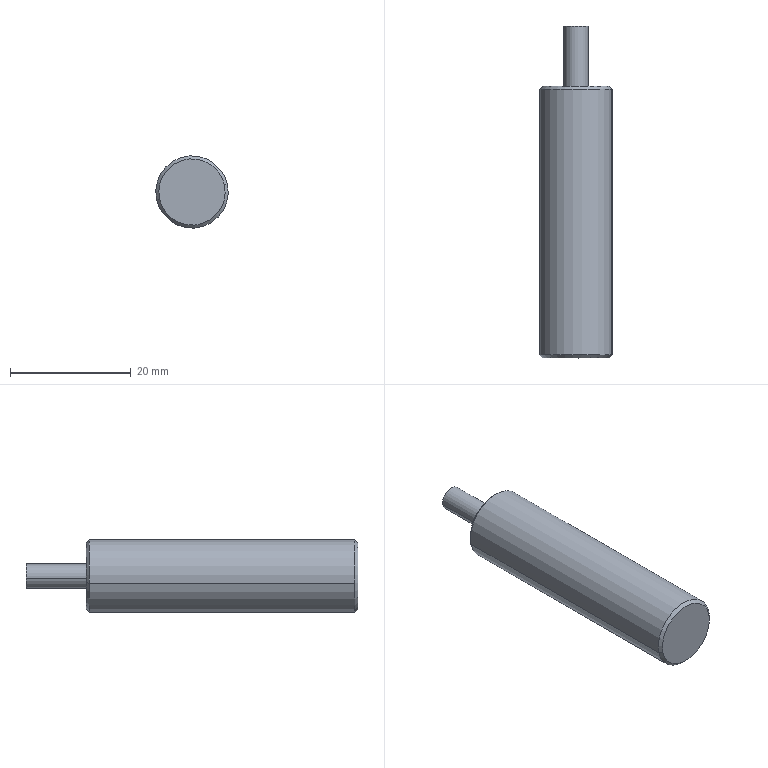Component | SolidWorks | ZJG28-1 | 1 solid | 11 faces | box 12 x 55 x 12 mm | volume 5206 mm3 | cone 4 | cylinder 4 | plane 3 | commonest cylinder face diameters 4 x2 12 x2
build123d program:
from build123d import *

# Parameters (mm, degrees)
SKETCH1_R           = 6
BOSS_EXTRUDE1_DEPTH = 45
SKETCH2_R           = 2
BOSS_EXTRUDE2_DEPTH = 10
CHAMFER1_SIZE       = 0.5


with BuildPart() as part:
    # Sketch1 → Boss-Extrude1 (new body)
    with BuildSketch(Plane.XY):
        with Locations(Location((0, 0, 0), (0, 0, 180))):
            Circle(SKETCH1_R)
    extrude(amount=BOSS_EXTRUDE1_DEPTH)

    # Sketch2 → Boss-Extrude2 (add)
    with BuildSketch(Plane.XY.offset(45)):
        Circle(SKETCH2_R)
    extrude(amount=BOSS_EXTRUDE2_DEPTH)

    # Chamfer1
    chamfer1_edges = [part.edges().sort_by_distance(p)[0] for p in [
        (6, 0, 0),
        (6, 0, 45),
    ]]
    chamfer(chamfer1_edges, length=CHAMFER1_SIZE)


solid = part.part

# Placed as in the assembly
solid = solid.moved(Location((-2.001, 46.001, -400), (-90, 0, 0)))
STEP:
#1=COLOUR_RGB('',0.7922,0.8196,0.9333);
#2=FILL_AREA_STYLE_COLOUR('',#1);
#3=FILL_AREA_STYLE('',(#2));
#4=SURFACE_STYLE_FILL_AREA(#3);
#5=SURFACE_SIDE_STYLE('',(#4));
#6=SURFACE_STYLE_USAGE(.BOTH.,#5);
#7=PRESENTATION_STYLE_ASSIGNMENT((#6));
#8=CARTESIAN_POINT('',(-0.2908,1.811,-15.792));
#9=VERTEX_POINT('',#8);
#10=CARTESIAN_POINT('',(0.1333,1.811,-15.704));
#11=VERTEX_POINT('',#10);
#12=CARTESIAN_POINT('',(-0.07876,1.811,-15.748));
#13=DIRECTION('',(0.,-1.,0.));
#14=DIRECTION('',(0.9793,0.,0.2022));
#15=AXIS2_PLACEMENT_3D('',#12,#13,#14);
#16=CIRCLE('',#15,0.2165);
#17=EDGE_CURVE('',#9,#11,#16,.T.);
#18=ORIENTED_EDGE('',*,*,#17,.F.);
#19=CARTESIAN_POINT('',(-0.3101,1.831,-15.796));
#20=VERTEX_POINT('',#19);
#21=CARTESIAN_POINT('',(-0.3101,1.831,-15.796));
#22=DIRECTION('',(-0.6925,0.7071,-0.143));
#23=VECTOR('',#22,39.37);
#24=LINE('',#21,#23);
#25=EDGE_CURVE('',#9,#20,#24,.T.);
#26=ORIENTED_EDGE('',*,*,#25,.T.);
#27=CARTESIAN_POINT('',(0.1526,1.831,-15.7));
#28=VERTEX_POINT('',#27);
#29=CARTESIAN_POINT('',(-0.07876,1.831,-15.748));
#30=DIRECTION('',(-0.,1.,-0.));
#31=DIRECTION('',(0.9793,0.,0.2022));
#32=AXIS2_PLACEMENT_3D('',#29,#30,#31);
#33=CIRCLE('',#32,0.2362);
#34=EDGE_CURVE('',#28,#20,#33,.T.);
#35=ORIENTED_EDGE('',*,*,#34,.F.);
#36=CARTESIAN_POINT('',(0.1526,1.831,-15.7));
#37=DIRECTION('',(0.6925,0.7071,0.143));
#38=VECTOR('',#37,39.37);
#39=LINE('',#36,#38);
#40=EDGE_CURVE('',#11,#28,#39,.T.);
#41=ORIENTED_EDGE('',*,*,#40,.F.);
#42=EDGE_LOOP('',(#18,#26,#35,#41));
#43=FACE_OUTER_BOUND('',#42,.T.);
#44=CARTESIAN_POINT('',(-0.07876,1.831,-15.748));
#45=DIRECTION('',(-0.,1.,-0.));
#46=DIRECTION('',(0.9793,0.,0.2022));
#47=AXIS2_PLACEMENT_3D('',#44,#45,#46);
#48=CONICAL_SURFACE('',#47,0.2362,0.7854);
#49=ADVANCED_FACE('',(#43),#48,.T.);
#50=CARTESIAN_POINT('',(0.1333,3.583,-15.704));
#51=VERTEX_POINT('',#50);
#52=CARTESIAN_POINT('',(-0.2908,3.583,-15.792));
#53=VERTEX_POINT('',#52);
#54=CARTESIAN_POINT('',(-0.07876,3.583,-15.748));
#55=DIRECTION('',(-0.,1.,-0.));
#56=DIRECTION('',(0.9793,0.,0.2022));
#57=AXIS2_PLACEMENT_3D('',#54,#55,#56);
#58=CIRCLE('',#57,0.2165);
#59=EDGE_CURVE('',#51,#53,#58,.T.);
#60=ORIENTED_EDGE('',*,*,#59,.F.);
#61=CARTESIAN_POINT('',(0.1526,3.563,-15.7));
#62=VERTEX_POINT('',#61);
#63=CARTESIAN_POINT('',(0.1333,3.583,-15.704));
#64=DIRECTION('',(0.6925,-0.7071,0.143));
#65=VECTOR('',#64,39.37);
#66=LINE('',#63,#65);
#67=EDGE_CURVE('',#51,#62,#66,.T.);
#68=ORIENTED_EDGE('',*,*,#67,.T.);
#69=CARTESIAN_POINT('',(-0.3101,3.563,-15.796));
#70=VERTEX_POINT('',#69);
#71=CARTESIAN_POINT('',(-0.07876,3.563,-15.748));
#72=DIRECTION('',(0.,-1.,0.));
#73=DIRECTION('',(0.9793,0.,0.2022));
#74=AXIS2_PLACEMENT_3D('',#71,#72,#73);
#75=CIRCLE('',#74,0.2362);
#76=EDGE_CURVE('',#70,#62,#75,.T.);
#77=ORIENTED_EDGE('',*,*,#76,.F.);
#78=CARTESIAN_POINT('',(-0.2908,3.583,-15.792));
#79=DIRECTION('',(-0.6925,-0.7071,-0.143));
#80=VECTOR('',#79,39.37);
#81=LINE('',#78,#80);
#82=EDGE_CURVE('',#53,#70,#81,.T.);
#83=ORIENTED_EDGE('',*,*,#82,.F.);
#84=EDGE_LOOP('',(#60,#68,#77,#83));
#85=FACE_OUTER_BOUND('',#84,.T.);
#86=CARTESIAN_POINT('',(-0.07876,3.583,-15.748));
#87=DIRECTION('',(0.,-1.,0.));
#88=DIRECTION('',(-0.9793,0.,-0.2022));
#89=AXIS2_PLACEMENT_3D('',#86,#87,#88);
#90=CONICAL_SURFACE('',#89,0.2165,0.7854);
#91=ADVANCED_FACE('',(#85),#90,.T.);
#92=CARTESIAN_POINT('',(-0.001647,3.976,-15.732));
#93=VERTEX_POINT('',#92);
#94=CARTESIAN_POINT('',(-0.1559,3.976,-15.764));
#95=VERTEX_POINT('',#94);
#96=CARTESIAN_POINT('',(-0.07876,3.976,-15.748));
#97=DIRECTION('',(-0.,1.,-0.));
#98=DIRECTION('',(0.9793,0.,0.2022));
#99=AXIS2_PLACEMENT_3D('',#96,#97,#98);
#100=CIRCLE('',#99,0.07874);
#101=EDGE_CURVE('',#93,#95,#100,.T.);
#102=ORIENTED_EDGE('',*,*,#101,.F.);
#103=CARTESIAN_POINT('',(-0.001647,3.583,-15.732));
#104=VERTEX_POINT('',#103);
#105=CARTESIAN_POINT('',(-0.001647,3.976,-15.732));
#106=DIRECTION('',(0.,-1.,0.));
#107=VECTOR('',#106,39.37);
#108=LINE('',#105,#107);
#109=EDGE_CURVE('',#93,#104,#108,.T.);
#110=ORIENTED_EDGE('',*,*,#109,.T.);
#111=CARTESIAN_POINT('',(-0.1559,3.583,-15.764));
#112=VERTEX_POINT('',#111);
#113=CARTESIAN_POINT('',(-0.07876,3.583,-15.748));
#114=DIRECTION('',(-0.,1.,-0.));
#115=DIRECTION('',(0.9793,0.,0.2022));
#116=AXIS2_PLACEMENT_3D('',#113,#114,#115);
#117=CIRCLE('',#116,0.07874);
#118=EDGE_CURVE('',#104,#112,#117,.T.);
#119=ORIENTED_EDGE('',*,*,#118,.T.);
#120=CARTESIAN_POINT('',(-0.1559,3.976,-15.764));
#121=DIRECTION('',(0.,-1.,0.));
#122=VECTOR('',#121,39.37);
#123=LINE('',#120,#122);
#124=EDGE_CURVE('',#95,#112,#123,.T.);
#125=ORIENTED_EDGE('',*,*,#124,.F.);
#126=EDGE_LOOP('',(#102,#110,#119,#125));
#127=FACE_OUTER_BOUND('',#126,.T.);
#128=CARTESIAN_POINT('',(-0.07876,3.976,-15.748));
#129=DIRECTION('',(0.,-1.,0.));
#130=DIRECTION('',(-0.9793,0.,-0.2022));
#131=AXIS2_PLACEMENT_3D('',#128,#129,#130);
#132=CYLINDRICAL_SURFACE('',#131,0.07874);
#133=ADVANCED_FACE('',(#127),#132,.T.);
#134=ORIENTED_EDGE('',*,*,#76,.T.);
#135=CARTESIAN_POINT('',(0.1526,3.583,-15.7));
#136=DIRECTION('',(0.,-1.,0.));
#137=VECTOR('',#136,39.37);
#138=LINE('',#135,#137);
#139=EDGE_CURVE('',#62,#28,#138,.T.);
#140=ORIENTED_EDGE('',*,*,#139,.T.);
#141=ORIENTED_EDGE('',*,*,#34,.T.);
#142=CARTESIAN_POINT('',(-0.3101,3.583,-15.796));
#143=DIRECTION('',(0.,-1.,0.));
#144=VECTOR('',#143,39.37);
#145=LINE('',#142,#144);
#146=EDGE_CURVE('',#70,#20,#145,.T.);
#147=ORIENTED_EDGE('',*,*,#146,.F.);
#148=EDGE_LOOP('',(#134,#140,#141,#147));
#149=FACE_OUTER_BOUND('',#148,.T.);
#150=CARTESIAN_POINT('',(-0.07876,3.583,-15.748));
#151=DIRECTION('',(0.,-1.,0.));
#152=DIRECTION('',(-0.9793,0.,-0.2022));
#153=AXIS2_PLACEMENT_3D('',#150,#151,#152);
#154=CYLINDRICAL_SURFACE('',#153,0.2362);
#155=ADVANCED_FACE('',(#149),#154,.T.);
#156=ORIENTED_EDGE('',*,*,#139,.F.);
#157=CARTESIAN_POINT('',(-0.07876,3.563,-15.748));
#158=DIRECTION('',(0.,-1.,0.));
#159=DIRECTION('',(0.9793,0.,0.2022));
#160=AXIS2_PLACEMENT_3D('',#157,#158,#159);
#161=CIRCLE('',#160,0.2362);
#162=EDGE_CURVE('',#62,#70,#161,.T.);
#163=ORIENTED_EDGE('',*,*,#162,.T.);
#164=ORIENTED_EDGE('',*,*,#146,.T.);
#165=CARTESIAN_POINT('',(-0.07876,1.831,-15.748));
#166=DIRECTION('',(-0.,1.,-0.));
#167=DIRECTION('',(0.9793,0.,0.2022));
#168=AXIS2_PLACEMENT_3D('',#165,#166,#167);
#169=CIRCLE('',#168,0.2362);
#170=EDGE_CURVE('',#20,#28,#169,.T.);
#171=ORIENTED_EDGE('',*,*,#170,.T.);
#172=EDGE_LOOP('',(#156,#163,#164,#171));
#173=FACE_OUTER_BOUND('',#172,.T.);
#174=CARTESIAN_POINT('',(-0.07876,3.583,-15.748));
#175=DIRECTION('',(0.,-1.,0.));
#176=DIRECTION('',(-0.9793,0.,-0.2022));
#177=AXIS2_PLACEMENT_3D('',#174,#175,#176);
#178=CYLINDRICAL_SURFACE('',#177,0.2362);
#179=ADVANCED_FACE('',(#173),#178,.T.);
#180=CARTESIAN_POINT('',(-0.07876,3.583,-15.748));
#181=DIRECTION('',(-0.,1.,-0.));
#182=DIRECTION('',(0.9793,0.,0.2022));
#183=AXIS2_PLACEMENT_3D('',#180,#181,#182);
#184=CIRCLE('',#183,0.2165);
#185=EDGE_CURVE('',#53,#51,#184,.T.);
#186=ORIENTED_EDGE('',*,*,#185,.T.);
#187=ORIENTED_EDGE('',*,*,#59,.T.);
#188=EDGE_LOOP('',(#186,#187));
#189=FACE_OUTER_BOUND('',#188,.T.);
#190=CARTESIAN_POINT('',(-0.07876,3.583,-15.748));
#191=DIRECTION('',(-0.,1.,-0.));
#192=DIRECTION('',(0.9793,0.,0.2022));
#193=AXIS2_PLACEMENT_3D('',#190,#191,#192);
#194=CIRCLE('',#193,0.07874);
#195=EDGE_CURVE('',#112,#104,#194,.T.);
#196=ORIENTED_EDGE('',*,*,#195,.F.);
#197=ORIENTED_EDGE('',*,*,#118,.F.);
#198=EDGE_LOOP('',(#196,#197));
#199=FACE_BOUND('',#198,.T.);
#200=CARTESIAN_POINT('',(-0.07876,3.583,-15.748));
#201=DIRECTION('',(-0.,1.,-0.));
#202=DIRECTION('',(0.9793,0.,0.2022));
#203=AXIS2_PLACEMENT_3D('',#200,#201,#202);
#204=PLANE('',#203);
#205=ADVANCED_FACE('',(#189,#199),#204,.T.);
#206=CARTESIAN_POINT('',(-0.07876,1.811,-15.748));
#207=DIRECTION('',(0.,-1.,0.));
#208=DIRECTION('',(0.9793,0.,0.2022));
#209=AXIS2_PLACEMENT_3D('',#206,#207,#208);
#210=CIRCLE('',#209,0.2165);
#211=EDGE_CURVE('',#11,#9,#210,.T.);
#212=ORIENTED_EDGE('',*,*,#211,.T.);
#213=ORIENTED_EDGE('',*,*,#17,.T.);
#214=EDGE_LOOP('',(#212,#213));
#215=FACE_OUTER_BOUND('',#214,.T.);
#216=CARTESIAN_POINT('',(-0.07876,1.811,-15.748));
#217=DIRECTION('',(-0.,1.,-0.));
#218=DIRECTION('',(0.9793,0.,0.2022));
#219=AXIS2_PLACEMENT_3D('',#216,#217,#218);
#220=PLANE('',#219);
#221=ADVANCED_FACE('',(#215),#220,.F.);
#222=ORIENTED_EDGE('',*,*,#109,.F.);
#223=CARTESIAN_POINT('',(-0.07876,3.976,-15.748));
#224=DIRECTION('',(-0.,1.,-0.));
#225=DIRECTION('',(0.9793,0.,0.2022));
#226=AXIS2_PLACEMENT_3D('',#223,#224,#225);
#227=CIRCLE('',#226,0.07874);
#228=EDGE_CURVE('',#95,#93,#227,.T.);
#229=ORIENTED_EDGE('',*,*,#228,.F.);
#230=ORIENTED_EDGE('',*,*,#124,.T.);
#231=ORIENTED_EDGE('',*,*,#195,.T.);
#232=EDGE_LOOP('',(#222,#229,#230,#231));
#233=FACE_OUTER_BOUND('',#232,.T.);
#234=CARTESIAN_POINT('',(-0.07876,3.976,-15.748));
#235=DIRECTION('',(0.,-1.,0.));
#236=DIRECTION('',(-0.9793,0.,-0.2022));
#237=AXIS2_PLACEMENT_3D('',#234,#235,#236);
#238=CYLINDRICAL_SURFACE('',#237,0.07874);
#239=ADVANCED_FACE('',(#233),#238,.T.);
#240=ORIENTED_EDGE('',*,*,#228,.T.);
#241=ORIENTED_EDGE('',*,*,#101,.T.);
#242=EDGE_LOOP('',(#240,#241));
#243=FACE_OUTER_BOUND('',#242,.T.);
#244=CARTESIAN_POINT('',(-0.07876,3.976,-15.748));
#245=DIRECTION('',(-0.,1.,-0.));
#246=DIRECTION('',(0.9793,0.,0.2022));
#247=AXIS2_PLACEMENT_3D('',#244,#245,#246);
#248=PLANE('',#247);
#249=ADVANCED_FACE('',(#243),#248,.T.);
#250=ORIENTED_EDGE('',*,*,#67,.F.);
#251=ORIENTED_EDGE('',*,*,#185,.F.);
#252=ORIENTED_EDGE('',*,*,#82,.T.);
#253=ORIENTED_EDGE('',*,*,#162,.F.);
#254=EDGE_LOOP('',(#250,#251,#252,#253));
#255=FACE_OUTER_BOUND('',#254,.T.);
#256=CARTESIAN_POINT('',(-0.07876,3.583,-15.748));
#257=DIRECTION('',(0.,-1.,0.));
#258=DIRECTION('',(-0.9793,0.,-0.2022));
#259=AXIS2_PLACEMENT_3D('',#256,#257,#258);
#260=CONICAL_SURFACE('',#259,0.2165,0.7854);
#261=ADVANCED_FACE('',(#255),#260,.T.);
#262=ORIENTED_EDGE('',*,*,#25,.F.);
#263=ORIENTED_EDGE('',*,*,#211,.F.);
#264=ORIENTED_EDGE('',*,*,#40,.T.);
#265=ORIENTED_EDGE('',*,*,#170,.F.);
#266=EDGE_LOOP('',(#262,#263,#264,#265));
#267=FACE_OUTER_BOUND('',#266,.T.);
#268=CARTESIAN_POINT('',(-0.07876,1.831,-15.748));
#269=DIRECTION('',(-0.,1.,-0.));
#270=DIRECTION('',(0.9793,0.,0.2022));
#271=AXIS2_PLACEMENT_3D('',#268,#269,#270);
#272=CONICAL_SURFACE('',#271,0.2362,0.7854);
#273=ADVANCED_FACE('',(#267),#272,.T.);
#274=CLOSED_SHELL('',(#49,#91,#133,#155,#179,#205,#221,#239,#249,#261,#273));
#275=MANIFOLD_SOLID_BREP('',#274);
#276=STYLED_ITEM('',(#7),#275);
#277=(LENGTH_UNIT()NAMED_UNIT(*)SI_UNIT($,.METRE.));
#278=LENGTH_MEASURE_WITH_UNIT(LENGTH_MEASURE(0.0254),#277);
#279=DIMENSIONAL_EXPONENTS(1.,0.,0.,0.,0.,0.,0.);
#280=(CONVERSION_BASED_UNIT('',#278)LENGTH_UNIT()NAMED_UNIT(#279));
#281=UNCERTAINTY_MEASURE_WITH_UNIT(LENGTH_MEASURE(0.00001),#280,'','');
#282=(NAMED_UNIT(*)PLANE_ANGLE_UNIT()SI_UNIT($,.RADIAN.));
#283=(NAMED_UNIT(*)SI_UNIT($,.STERADIAN.)SOLID_ANGLE_UNIT());
#284=(GEOMETRIC_REPRESENTATION_CONTEXT(3)GLOBAL_UNCERTAINTY_ASSIGNED_CONTEXT((#281))GLOBAL_UNIT_ASSIGNED_CONTEXT((#280,#282,#283))REPRESENTATION_CONTEXT('',''));
#285=MECHANICAL_DESIGN_GEOMETRIC_PRESENTATION_REPRESENTATION('',(#276),#284);
#286=PRESENTATION_LAYER_ASSIGNMENT('','',(#276));
#287=CARTESIAN_POINT('',(0.,0.,0.));
#288=DIRECTION('',(0.,0.,1.));
#289=DIRECTION('',(1.,0.,0.));
#290=AXIS2_PLACEMENT_3D('',#287,#288,#289);
#291=(LENGTH_UNIT()NAMED_UNIT(*)SI_UNIT($,.METRE.));
#292=LENGTH_MEASURE_WITH_UNIT(LENGTH_MEASURE(0.0254),#291);
#293=DIMENSIONAL_EXPONENTS(1.,0.,0.,0.,0.,0.,0.);
#294=(CONVERSION_BASED_UNIT('',#292)LENGTH_UNIT()NAMED_UNIT(#293));
#295=UNCERTAINTY_MEASURE_WITH_UNIT(LENGTH_MEASURE(0.00001),#294,'','');
#296=(NAMED_UNIT(*)PLANE_ANGLE_UNIT()SI_UNIT($,.RADIAN.));
#297=(NAMED_UNIT(*)SI_UNIT($,.STERADIAN.)SOLID_ANGLE_UNIT());
#298=(GEOMETRIC_REPRESENTATION_CONTEXT(3)GLOBAL_UNCERTAINTY_ASSIGNED_CONTEXT((#295))GLOBAL_UNIT_ASSIGNED_CONTEXT((#294,#296,#297))REPRESENTATION_CONTEXT('',''));
#299=ADVANCED_BREP_SHAPE_REPRESENTATION('',(#275,#290),#298);